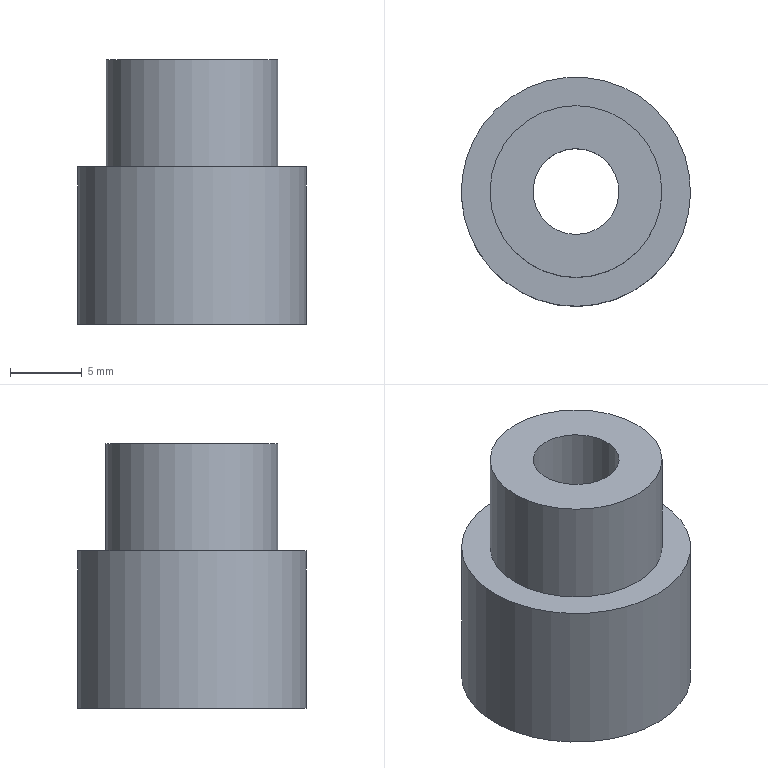Component | NX | 05C__27 | 1 solid | 8 faces | box 16 x 16 x 18.5 mm | volume 1590 mm3 | cylinder 4 | plane 3 | cone 1 | commonest cylinder face diameters 12 x2 6 x1 16 x1
STEP:
#1=CARTESIAN_POINT('',(0.,0.,0.));
#2=DIRECTION('',(0.,0.,1.));
#3=DIRECTION('',(1.,0.,0.));
#4=AXIS2_PLACEMENT_3D('',#1,#2,#3);
#5=CARTESIAN_POINT('',(73.251,108.441,194.432));
#6=VERTEX_POINT('',#5);
#7=CARTESIAN_POINT('',(76.022,109.59,194.432));
#8=DIRECTION('',(0.,0.,1.));
#9=DIRECTION('',(-0.9237,-0.383,0.));
#10=AXIS2_PLACEMENT_3D('',#7,#8,#9);
#11=CIRCLE('',#10,3.);
#12=CARTESIAN_POINT('',(76.022,109.59,194.432));
#13=DIRECTION('',(0.,0.,1.));
#14=DIRECTION('',(-0.9237,-0.383,0.));
#15=AXIS2_PLACEMENT_3D('',#12,#13,#14);
#16=CYLINDRICAL_SURFACE('',#15,3.);
#17=CARTESIAN_POINT('',(0.,0.));
#18=DIRECTION('',(1.,0.));
#19=VECTOR('',#18,1.);
#20=LINE('',#17,#19);
#21=(GEOMETRIC_REPRESENTATION_CONTEXT(2)PARAMETRIC_REPRESENTATION_CONTEXT()REPRESENTATION_CONTEXT('',''));
#22=DEFINITIONAL_REPRESENTATION('',(#20),#21);
#23=PCURVE('',#16,#22);
#24=CARTESIAN_POINT('',(77.171,106.819,194.432));
#25=DIRECTION('',(0.,0.,1.));
#26=DIRECTION('',(-0.9237,-0.383,0.));
#27=AXIS2_PLACEMENT_3D('',#24,#25,#26);
#28=PLANE('',#27);
#29=CARTESIAN_POINT('',(0.,-3.));
#30=DIRECTION('',(1.,-0.));
#31=AXIS2_PLACEMENT_2D('',#29,#30);
#32=CIRCLE('',#31,3.);
#33=(GEOMETRIC_REPRESENTATION_CONTEXT(2)PARAMETRIC_REPRESENTATION_CONTEXT()REPRESENTATION_CONTEXT('',''));
#34=DEFINITIONAL_REPRESENTATION('',(#32),#33);
#35=PCURVE('',#28,#34);
#36=SURFACE_CURVE('',#11,(#23,#35),.PCURVE_S1.);
#37=EDGE_CURVE('',#6,#6,#36,.T.);
#38=ORIENTED_EDGE('',*,*,#37,.F.);
#39=CARTESIAN_POINT('',(73.251,108.441,187.932));
#40=VERTEX_POINT('',#39);
#41=CARTESIAN_POINT('',(73.251,108.441,187.932));
#42=CARTESIAN_POINT('',(73.251,108.441,194.432));
#43=B_SPLINE_CURVE_WITH_KNOTS('',1,(#41,#42),.UNSPECIFIED.,.F.,.F.,(2,2),(-6.5,0.),.PIECEWISE_BEZIER_KNOTS.);
#44=CARTESIAN_POINT('',(0.,0.));
#45=DIRECTION('',(0.,1.));
#46=VECTOR('',#45,1.);
#47=LINE('',#44,#46);
#48=(GEOMETRIC_REPRESENTATION_CONTEXT(2)PARAMETRIC_REPRESENTATION_CONTEXT()REPRESENTATION_CONTEXT('',''));
#49=DEFINITIONAL_REPRESENTATION('',(#47),#48);
#50=PCURVE('',#16,#49);
#51=CARTESIAN_POINT('',(6.283,0.));
#52=DIRECTION('',(0.,1.));
#53=VECTOR('',#52,1.);
#54=LINE('',#51,#53);
#55=(GEOMETRIC_REPRESENTATION_CONTEXT(2)PARAMETRIC_REPRESENTATION_CONTEXT()REPRESENTATION_CONTEXT('',''));
#56=DEFINITIONAL_REPRESENTATION('',(#54),#55);
#57=PCURVE('',#16,#56);
#58=SEAM_CURVE('',#43,(#50,#57),.PCURVE_S1.);
#59=EDGE_CURVE('',#40,#6,#58,.T.);
#60=ORIENTED_EDGE('',*,*,#59,.F.);
#61=CARTESIAN_POINT('',(76.022,109.59,187.932));
#62=DIRECTION('',(0.,0.,1.));
#63=DIRECTION('',(-0.9237,-0.383,0.));
#64=AXIS2_PLACEMENT_3D('',#61,#62,#63);
#65=CIRCLE('',#64,3.);
#66=CARTESIAN_POINT('',(0.,-6.5));
#67=DIRECTION('',(1.,0.));
#68=VECTOR('',#67,1.);
#69=LINE('',#66,#68);
#70=(GEOMETRIC_REPRESENTATION_CONTEXT(2)PARAMETRIC_REPRESENTATION_CONTEXT()REPRESENTATION_CONTEXT('',''));
#71=DEFINITIONAL_REPRESENTATION('',(#69),#70);
#72=PCURVE('',#16,#71);
#73=CARTESIAN_POINT('',(76.022,109.59,186.432));
#74=DIRECTION('',(0.,0.,-1.));
#75=DIRECTION('',(0.9237,0.383,0.));
#76=AXIS2_PLACEMENT_3D('',#73,#74,#75);
#77=CONICAL_SURFACE('',#76,6.,1.107);
#78=CARTESIAN_POINT('',(9.425,-1.5));
#79=DIRECTION('',(-1.,0.));
#80=VECTOR('',#79,1.);
#81=LINE('',#78,#80);
#82=(GEOMETRIC_REPRESENTATION_CONTEXT(2)PARAMETRIC_REPRESENTATION_CONTEXT()REPRESENTATION_CONTEXT('',''));
#83=DEFINITIONAL_REPRESENTATION('',(#81),#82);
#84=PCURVE('',#77,#83);
#85=SURFACE_CURVE('',#65,(#72,#84),.PCURVE_S1.);
#86=EDGE_CURVE('',#40,#40,#85,.T.);
#87=ORIENTED_EDGE('',*,*,#86,.T.);
#88=ORIENTED_EDGE('',*,*,#59,.T.);
#89=EDGE_LOOP('',(#38,#60,#87,#88));
#90=FACE_BOUND('',#89,.F.);
#91=ADVANCED_FACE('',(#90),#16,.F.);
#92=CARTESIAN_POINT('',(70.48,107.292,194.432));
#93=VERTEX_POINT('',#92);
#94=CARTESIAN_POINT('',(76.022,109.59,194.432));
#95=DIRECTION('',(0.,0.,1.));
#96=DIRECTION('',(-0.9237,-0.383,0.));
#97=AXIS2_PLACEMENT_3D('',#94,#95,#96);
#98=CIRCLE('',#97,6.);
#99=CARTESIAN_POINT('',(0.,-3.));
#100=DIRECTION('',(1.,0.));
#101=AXIS2_PLACEMENT_2D('',#99,#100);
#102=CIRCLE('',#101,6.);
#103=(GEOMETRIC_REPRESENTATION_CONTEXT(2)PARAMETRIC_REPRESENTATION_CONTEXT()REPRESENTATION_CONTEXT('',''));
#104=DEFINITIONAL_REPRESENTATION('',(#102),#103);
#105=PCURVE('',#28,#104);
#106=CARTESIAN_POINT('',(76.022,109.59,194.432));
#107=DIRECTION('',(0.,0.,1.));
#108=DIRECTION('',(-0.9237,-0.383,0.));
#109=AXIS2_PLACEMENT_3D('',#106,#107,#108);
#110=CYLINDRICAL_SURFACE('',#109,6.);
#111=CARTESIAN_POINT('',(0.,0.));
#112=DIRECTION('',(1.,0.));
#113=VECTOR('',#112,1.);
#114=LINE('',#111,#113);
#115=(GEOMETRIC_REPRESENTATION_CONTEXT(2)PARAMETRIC_REPRESENTATION_CONTEXT()REPRESENTATION_CONTEXT('',''));
#116=DEFINITIONAL_REPRESENTATION('',(#114),#115);
#117=PCURVE('',#110,#116);
#118=SURFACE_CURVE('',#98,(#105,#117),.PCURVE_S1.);
#119=EDGE_CURVE('',#93,#93,#118,.T.);
#120=ORIENTED_EDGE('',*,*,#119,.T.);
#121=EDGE_LOOP('',(#120));
#122=FACE_BOUND('',#121,.T.);
#123=ORIENTED_EDGE('',*,*,#37,.F.);
#124=EDGE_LOOP('',(#123));
#125=FACE_BOUND('',#124,.T.);
#126=ADVANCED_FACE('',(#122,#125),#28,.T.);
#127=CARTESIAN_POINT('',(70.48,107.292,186.932));
#128=VERTEX_POINT('',#127);
#129=CARTESIAN_POINT('',(76.022,109.59,186.932));
#130=DIRECTION('',(0.,0.,1.));
#131=DIRECTION('',(-0.9237,-0.383,0.));
#132=AXIS2_PLACEMENT_3D('',#129,#130,#131);
#133=CIRCLE('',#132,6.);
#134=CARTESIAN_POINT('',(0.,-7.5));
#135=DIRECTION('',(1.,0.));
#136=VECTOR('',#135,1.);
#137=LINE('',#134,#136);
#138=(GEOMETRIC_REPRESENTATION_CONTEXT(2)PARAMETRIC_REPRESENTATION_CONTEXT()REPRESENTATION_CONTEXT('',''));
#139=DEFINITIONAL_REPRESENTATION('',(#137),#138);
#140=PCURVE('',#110,#139);
#141=CARTESIAN_POINT('',(78.32,104.048,186.932));
#142=DIRECTION('',(0.,0.,1.));
#143=DIRECTION('',(-0.9237,-0.383,0.));
#144=AXIS2_PLACEMENT_3D('',#141,#142,#143);
#145=PLANE('',#144);
#146=CARTESIAN_POINT('',(-0.,-6.));
#147=DIRECTION('',(1.,-0.));
#148=AXIS2_PLACEMENT_2D('',#146,#147);
#149=CIRCLE('',#148,6.);
#150=(GEOMETRIC_REPRESENTATION_CONTEXT(2)PARAMETRIC_REPRESENTATION_CONTEXT()REPRESENTATION_CONTEXT('',''));
#151=DEFINITIONAL_REPRESENTATION('',(#149),#150);
#152=PCURVE('',#145,#151);
#153=SURFACE_CURVE('',#133,(#140,#152),.PCURVE_S1.);
#154=EDGE_CURVE('',#128,#128,#153,.T.);
#155=ORIENTED_EDGE('',*,*,#154,.T.);
#156=CARTESIAN_POINT('',(70.48,107.292,186.932));
#157=CARTESIAN_POINT('',(70.48,107.292,194.432));
#158=B_SPLINE_CURVE_WITH_KNOTS('',1,(#156,#157),.UNSPECIFIED.,.F.,.F.,(2,2),(-7.5,0.),.PIECEWISE_BEZIER_KNOTS.);
#159=CARTESIAN_POINT('',(6.283,0.));
#160=DIRECTION('',(0.,1.));
#161=VECTOR('',#160,1.);
#162=LINE('',#159,#161);
#163=(GEOMETRIC_REPRESENTATION_CONTEXT(2)PARAMETRIC_REPRESENTATION_CONTEXT()REPRESENTATION_CONTEXT('',''));
#164=DEFINITIONAL_REPRESENTATION('',(#162),#163);
#165=PCURVE('',#110,#164);
#166=CARTESIAN_POINT('',(0.,0.));
#167=DIRECTION('',(0.,1.));
#168=VECTOR('',#167,1.);
#169=LINE('',#166,#168);
#170=(GEOMETRIC_REPRESENTATION_CONTEXT(2)PARAMETRIC_REPRESENTATION_CONTEXT()REPRESENTATION_CONTEXT('',''));
#171=DEFINITIONAL_REPRESENTATION('',(#169),#170);
#172=PCURVE('',#110,#171);
#173=SEAM_CURVE('',#158,(#165,#172),.PCURVE_S1.);
#174=EDGE_CURVE('',#128,#93,#173,.T.);
#175=ORIENTED_EDGE('',*,*,#174,.T.);
#176=ORIENTED_EDGE('',*,*,#119,.F.);
#177=ORIENTED_EDGE('',*,*,#174,.F.);
#178=EDGE_LOOP('',(#155,#175,#176,#177));
#179=FACE_BOUND('',#178,.T.);
#180=ADVANCED_FACE('',(#179),#110,.T.);
#181=CARTESIAN_POINT('',(68.632,106.526,186.932));
#182=VERTEX_POINT('',#181);
#183=CARTESIAN_POINT('',(76.022,109.59,186.932));
#184=DIRECTION('',(0.,0.,1.));
#185=DIRECTION('',(-0.9237,-0.383,0.));
#186=AXIS2_PLACEMENT_3D('',#183,#184,#185);
#187=CIRCLE('',#186,8.);
#188=CARTESIAN_POINT('',(-0.,-6.));
#189=DIRECTION('',(1.,-0.));
#190=AXIS2_PLACEMENT_2D('',#188,#189);
#191=CIRCLE('',#190,8.);
#192=(GEOMETRIC_REPRESENTATION_CONTEXT(2)PARAMETRIC_REPRESENTATION_CONTEXT()REPRESENTATION_CONTEXT('',''));
#193=DEFINITIONAL_REPRESENTATION('',(#191),#192);
#194=PCURVE('',#145,#193);
#195=CARTESIAN_POINT('',(76.022,109.59,194.432));
#196=DIRECTION('',(0.,0.,1.));
#197=DIRECTION('',(-0.9237,-0.383,0.));
#198=AXIS2_PLACEMENT_3D('',#195,#196,#197);
#199=CYLINDRICAL_SURFACE('',#198,8.);
#200=CARTESIAN_POINT('',(0.,-7.5));
#201=DIRECTION('',(1.,0.));
#202=VECTOR('',#201,1.);
#203=LINE('',#200,#202);
#204=(GEOMETRIC_REPRESENTATION_CONTEXT(2)PARAMETRIC_REPRESENTATION_CONTEXT()REPRESENTATION_CONTEXT('',''));
#205=DEFINITIONAL_REPRESENTATION('',(#203),#204);
#206=PCURVE('',#199,#205);
#207=SURFACE_CURVE('',#187,(#194,#206),.PCURVE_S1.);
#208=EDGE_CURVE('',#182,#182,#207,.T.);
#209=ORIENTED_EDGE('',*,*,#208,.T.);
#210=EDGE_LOOP('',(#209));
#211=FACE_BOUND('',#210,.T.);
#212=ORIENTED_EDGE('',*,*,#154,.F.);
#213=EDGE_LOOP('',(#212));
#214=FACE_BOUND('',#213,.T.);
#215=ADVANCED_FACE('',(#211,#214),#145,.T.);
#216=CARTESIAN_POINT('',(68.632,106.526,175.932));
#217=VERTEX_POINT('',#216);
#218=CARTESIAN_POINT('',(76.022,109.59,175.932));
#219=DIRECTION('',(0.,0.,1.));
#220=DIRECTION('',(-0.9237,-0.383,0.));
#221=AXIS2_PLACEMENT_3D('',#218,#219,#220);
#222=CIRCLE('',#221,8.);
#223=CARTESIAN_POINT('',(0.,-18.5));
#224=DIRECTION('',(1.,0.));
#225=VECTOR('',#224,1.);
#226=LINE('',#223,#225);
#227=(GEOMETRIC_REPRESENTATION_CONTEXT(2)PARAMETRIC_REPRESENTATION_CONTEXT()REPRESENTATION_CONTEXT('',''));
#228=DEFINITIONAL_REPRESENTATION('',(#226),#227);
#229=PCURVE('',#199,#228);
#230=CARTESIAN_POINT('',(79.087,102.2,175.932));
#231=DIRECTION('',(0.,0.,-1.));
#232=DIRECTION('',(0.9237,0.383,0.));
#233=AXIS2_PLACEMENT_3D('',#230,#231,#232);
#234=PLANE('',#233);
#235=CARTESIAN_POINT('',(-8.,-8.));
#236=CARTESIAN_POINT('',(-8.,5.856));
#237=CARTESIAN_POINT('',(4.,-1.072));
#238=CARTESIAN_POINT('',(16.,-8.));
#239=CARTESIAN_POINT('',(4.,-14.928));
#240=CARTESIAN_POINT('',(-8.,-21.856));
#241=CARTESIAN_POINT('',(-8.,-8.));
#242=(BOUNDED_CURVE()B_SPLINE_CURVE(2,(#235,#236,#237,#238,#239,#240,#241),.UNSPECIFIED.,.T.,.F.)B_SPLINE_CURVE_WITH_KNOTS((1,2,2,2,2,1),(-2.094,0.,2.094,4.189,6.283,8.378),.UNSPECIFIED.)CURVE()GEOMETRIC_REPRESENTATION_ITEM()RATIONAL_B_SPLINE_CURVE((1.,0.5,1.,0.5,1.,0.5,1.))REPRESENTATION_ITEM(''));
#243=(GEOMETRIC_REPRESENTATION_CONTEXT(2)PARAMETRIC_REPRESENTATION_CONTEXT()REPRESENTATION_CONTEXT('',''));
#244=DEFINITIONAL_REPRESENTATION('',(#242),#243);
#245=PCURVE('',#234,#244);
#246=SURFACE_CURVE('',#222,(#229,#245),.PCURVE_S1.);
#247=EDGE_CURVE('',#217,#217,#246,.T.);
#248=ORIENTED_EDGE('',*,*,#247,.T.);
#249=CARTESIAN_POINT('',(68.632,106.526,175.932));
#250=CARTESIAN_POINT('',(68.632,106.526,186.932));
#251=B_SPLINE_CURVE_WITH_KNOTS('',1,(#249,#250),.UNSPECIFIED.,.F.,.F.,(2,2),(-18.5,-7.5),.PIECEWISE_BEZIER_KNOTS.);
#252=CARTESIAN_POINT('',(6.283,0.));
#253=DIRECTION('',(0.,1.));
#254=VECTOR('',#253,1.);
#255=LINE('',#252,#254);
#256=(GEOMETRIC_REPRESENTATION_CONTEXT(2)PARAMETRIC_REPRESENTATION_CONTEXT()REPRESENTATION_CONTEXT('',''));
#257=DEFINITIONAL_REPRESENTATION('',(#255),#256);
#258=PCURVE('',#199,#257);
#259=CARTESIAN_POINT('',(0.,0.));
#260=DIRECTION('',(0.,1.));
#261=VECTOR('',#260,1.);
#262=LINE('',#259,#261);
#263=(GEOMETRIC_REPRESENTATION_CONTEXT(2)PARAMETRIC_REPRESENTATION_CONTEXT()REPRESENTATION_CONTEXT('',''));
#264=DEFINITIONAL_REPRESENTATION('',(#262),#263);
#265=PCURVE('',#199,#264);
#266=SEAM_CURVE('',#251,(#258,#265),.PCURVE_S1.);
#267=EDGE_CURVE('',#217,#182,#266,.T.);
#268=ORIENTED_EDGE('',*,*,#267,.T.);
#269=ORIENTED_EDGE('',*,*,#208,.F.);
#270=ORIENTED_EDGE('',*,*,#267,.F.);
#271=EDGE_LOOP('',(#248,#268,#269,#270));
#272=FACE_BOUND('',#271,.T.);
#273=ADVANCED_FACE('',(#272),#199,.T.);
#274=CARTESIAN_POINT('',(70.48,107.292,175.932));
#275=VERTEX_POINT('',#274);
#276=CARTESIAN_POINT('',(76.022,109.59,175.932));
#277=DIRECTION('',(0.,0.,1.));
#278=DIRECTION('',(-0.9237,-0.383,0.));
#279=AXIS2_PLACEMENT_3D('',#276,#277,#278);
#280=CIRCLE('',#279,6.);
#281=CARTESIAN_POINT('',(-6.,-8.));
#282=CARTESIAN_POINT('',(-6.,2.392));
#283=CARTESIAN_POINT('',(3.,-2.804));
#284=CARTESIAN_POINT('',(12.,-8.));
#285=CARTESIAN_POINT('',(3.,-13.196));
#286=CARTESIAN_POINT('',(-6.,-18.392));
#287=CARTESIAN_POINT('',(-6.,-8.));
#288=(BOUNDED_CURVE()B_SPLINE_CURVE(2,(#281,#282,#283,#284,#285,#286,#287),.UNSPECIFIED.,.T.,.F.)B_SPLINE_CURVE_WITH_KNOTS((1,2,2,2,2,1),(-2.094,0.,2.094,4.189,6.283,8.378),.UNSPECIFIED.)CURVE()GEOMETRIC_REPRESENTATION_ITEM()RATIONAL_B_SPLINE_CURVE((1.,0.5,1.,0.5,1.,0.5,1.))REPRESENTATION_ITEM(''));
#289=(GEOMETRIC_REPRESENTATION_CONTEXT(2)PARAMETRIC_REPRESENTATION_CONTEXT()REPRESENTATION_CONTEXT('',''));
#290=DEFINITIONAL_REPRESENTATION('',(#288),#289);
#291=PCURVE('',#234,#290);
#292=CARTESIAN_POINT('',(76.022,109.59,194.432));
#293=DIRECTION('',(0.,0.,1.));
#294=DIRECTION('',(-0.9237,-0.383,0.));
#295=AXIS2_PLACEMENT_3D('',#292,#293,#294);
#296=CYLINDRICAL_SURFACE('',#295,6.);
#297=CARTESIAN_POINT('',(0.,-18.5));
#298=DIRECTION('',(1.,0.));
#299=VECTOR('',#298,1.);
#300=LINE('',#297,#299);
#301=(GEOMETRIC_REPRESENTATION_CONTEXT(2)PARAMETRIC_REPRESENTATION_CONTEXT()REPRESENTATION_CONTEXT('',''));
#302=DEFINITIONAL_REPRESENTATION('',(#300),#301);
#303=PCURVE('',#296,#302);
#304=SURFACE_CURVE('',#280,(#291,#303),.PCURVE_S1.);
#305=EDGE_CURVE('',#275,#275,#304,.T.);
#306=ORIENTED_EDGE('',*,*,#305,.T.);
#307=EDGE_LOOP('',(#306));
#308=FACE_BOUND('',#307,.T.);
#309=ORIENTED_EDGE('',*,*,#247,.F.);
#310=EDGE_LOOP('',(#309));
#311=FACE_BOUND('',#310,.T.);
#312=ADVANCED_FACE('',(#308,#311),#234,.T.);
#313=CARTESIAN_POINT('',(70.48,107.292,186.432));
#314=VERTEX_POINT('',#313);
#315=CARTESIAN_POINT('',(76.022,109.59,186.432));
#316=DIRECTION('',(0.,0.,1.));
#317=DIRECTION('',(-0.9237,-0.383,0.));
#318=AXIS2_PLACEMENT_3D('',#315,#316,#317);
#319=CIRCLE('',#318,6.);
#320=CARTESIAN_POINT('',(0.,-8.));
#321=DIRECTION('',(1.,0.));
#322=VECTOR('',#321,1.);
#323=LINE('',#320,#322);
#324=(GEOMETRIC_REPRESENTATION_CONTEXT(2)PARAMETRIC_REPRESENTATION_CONTEXT()REPRESENTATION_CONTEXT('',''));
#325=DEFINITIONAL_REPRESENTATION('',(#323),#324);
#326=PCURVE('',#296,#325);
#327=CARTESIAN_POINT('',(9.425,0.));
#328=DIRECTION('',(-1.,0.));
#329=VECTOR('',#328,1.);
#330=LINE('',#327,#329);
#331=(GEOMETRIC_REPRESENTATION_CONTEXT(2)PARAMETRIC_REPRESENTATION_CONTEXT()REPRESENTATION_CONTEXT('',''));
#332=DEFINITIONAL_REPRESENTATION('',(#330),#331);
#333=PCURVE('',#77,#332);
#334=SURFACE_CURVE('',#319,(#326,#333),.PCURVE_S1.);
#335=EDGE_CURVE('',#314,#314,#334,.T.);
#336=ORIENTED_EDGE('',*,*,#335,.F.);
#337=CARTESIAN_POINT('',(70.48,107.292,175.932));
#338=CARTESIAN_POINT('',(70.48,107.292,186.432));
#339=B_SPLINE_CURVE_WITH_KNOTS('',1,(#337,#338),.UNSPECIFIED.,.F.,.F.,(2,2),(-18.5,-8.),.PIECEWISE_BEZIER_KNOTS.);
#340=CARTESIAN_POINT('',(0.,0.));
#341=DIRECTION('',(0.,1.));
#342=VECTOR('',#341,1.);
#343=LINE('',#340,#342);
#344=(GEOMETRIC_REPRESENTATION_CONTEXT(2)PARAMETRIC_REPRESENTATION_CONTEXT()REPRESENTATION_CONTEXT('',''));
#345=DEFINITIONAL_REPRESENTATION('',(#343),#344);
#346=PCURVE('',#296,#345);
#347=CARTESIAN_POINT('',(6.283,0.));
#348=DIRECTION('',(0.,1.));
#349=VECTOR('',#348,1.);
#350=LINE('',#347,#349);
#351=(GEOMETRIC_REPRESENTATION_CONTEXT(2)PARAMETRIC_REPRESENTATION_CONTEXT()REPRESENTATION_CONTEXT('',''));
#352=DEFINITIONAL_REPRESENTATION('',(#350),#351);
#353=PCURVE('',#296,#352);
#354=SEAM_CURVE('',#339,(#346,#353),.PCURVE_S1.);
#355=EDGE_CURVE('',#275,#314,#354,.T.);
#356=ORIENTED_EDGE('',*,*,#355,.F.);
#357=ORIENTED_EDGE('',*,*,#305,.T.);
#358=ORIENTED_EDGE('',*,*,#355,.T.);
#359=EDGE_LOOP('',(#336,#356,#357,#358));
#360=FACE_BOUND('',#359,.F.);
#361=ADVANCED_FACE('',(#360),#296,.F.);
#362=ORIENTED_EDGE('',*,*,#86,.F.);
#363=CARTESIAN_POINT('',(73.251,108.441,187.932));
#364=CARTESIAN_POINT('',(70.48,107.292,186.432));
#365=B_SPLINE_CURVE_WITH_KNOTS('',1,(#363,#364),.UNSPECIFIED.,.F.,.F.,(2,2),(-3.354,0.),.PIECEWISE_BEZIER_KNOTS.);
#366=CARTESIAN_POINT('',(9.425,0.));
#367=DIRECTION('',(0.,1.));
#368=VECTOR('',#367,1.);
#369=LINE('',#366,#368);
#370=(GEOMETRIC_REPRESENTATION_CONTEXT(2)PARAMETRIC_REPRESENTATION_CONTEXT()REPRESENTATION_CONTEXT('',''));
#371=DEFINITIONAL_REPRESENTATION('',(#369),#370);
#372=PCURVE('',#77,#371);
#373=CARTESIAN_POINT('',(3.142,0.));
#374=DIRECTION('',(0.,1.));
#375=VECTOR('',#374,1.);
#376=LINE('',#373,#375);
#377=(GEOMETRIC_REPRESENTATION_CONTEXT(2)PARAMETRIC_REPRESENTATION_CONTEXT()REPRESENTATION_CONTEXT('',''));
#378=DEFINITIONAL_REPRESENTATION('',(#376),#377);
#379=PCURVE('',#77,#378);
#380=SEAM_CURVE('',#365,(#372,#379),.PCURVE_S1.);
#381=EDGE_CURVE('',#40,#314,#380,.T.);
#382=ORIENTED_EDGE('',*,*,#381,.T.);
#383=ORIENTED_EDGE('',*,*,#335,.T.);
#384=ORIENTED_EDGE('',*,*,#381,.F.);
#385=EDGE_LOOP('',(#362,#382,#383,#384));
#386=FACE_BOUND('',#385,.F.);
#387=ADVANCED_FACE('',(#386),#77,.F.);
#388=CLOSED_SHELL('',(#91,#126,#180,#215,#273,#312,#361,#387));
#389=MANIFOLD_SOLID_BREP('',#388);
#390=(LENGTH_UNIT()NAMED_UNIT(*)SI_UNIT(.MILLI.,.METRE.));
#391=UNCERTAINTY_MEASURE_WITH_UNIT(LENGTH_MEASURE(0.00001),#390,'','');
#392=(NAMED_UNIT(*)PLANE_ANGLE_UNIT()SI_UNIT($,.RADIAN.));
#393=(NAMED_UNIT(*)SI_UNIT($,.STERADIAN.)SOLID_ANGLE_UNIT());
#394=(GEOMETRIC_REPRESENTATION_CONTEXT(3)GLOBAL_UNCERTAINTY_ASSIGNED_CONTEXT((#391))GLOBAL_UNIT_ASSIGNED_CONTEXT((#390,#392,#393))REPRESENTATION_CONTEXT('',''));
#395=ADVANCED_BREP_SHAPE_REPRESENTATION('',(#4,#389),#394);